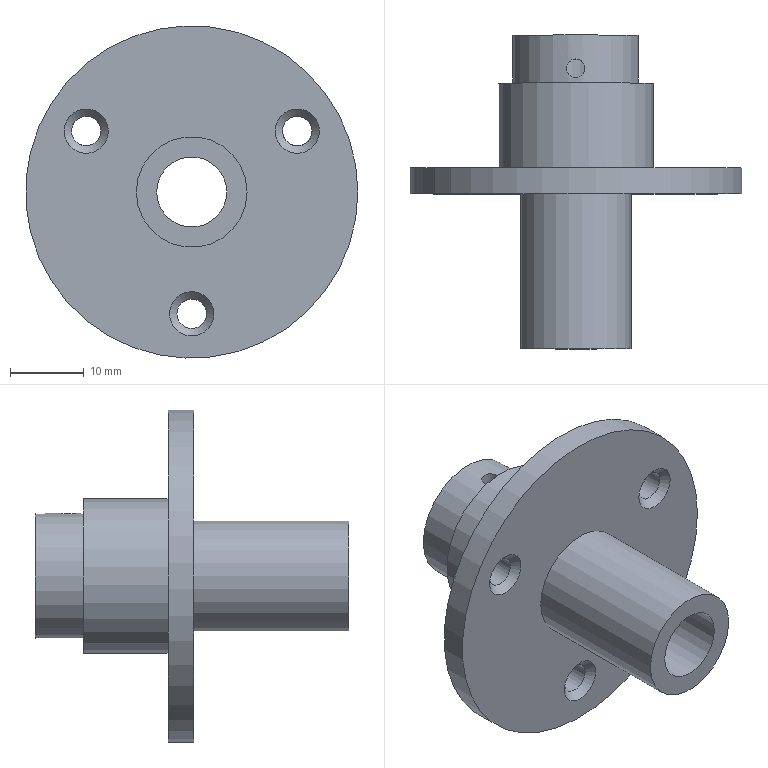Component | NX | FLYWHEEL_SHAFT | 1 solid | 17 faces | volume 11551 mm3 | cylinder 9 | plane 5 | cone 3 | commonest cylinder face diameters 4 x3 17 x1 21 x1 45 x1 15 x1 9.5 x1 2.5 x1